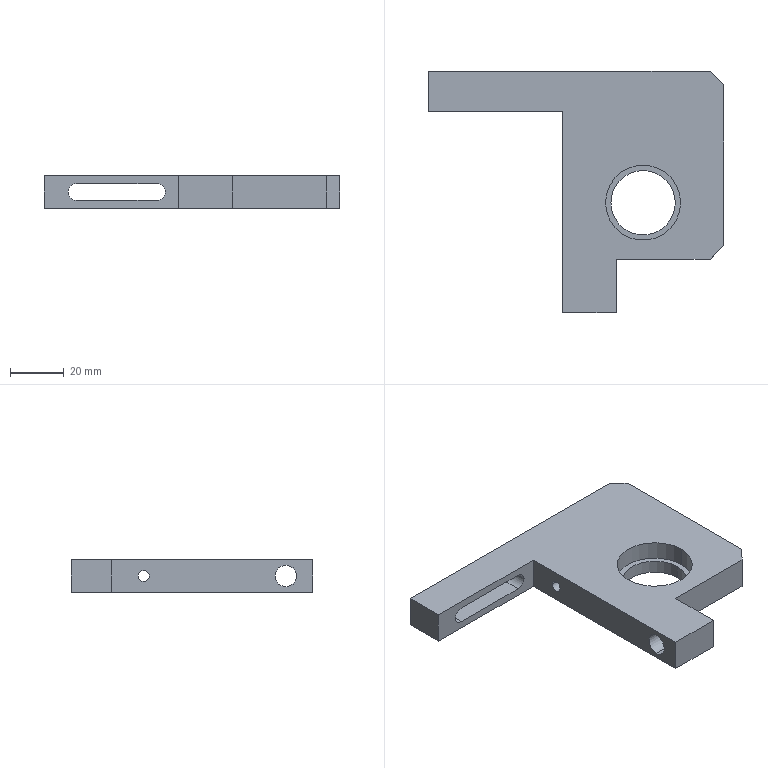Component | SolidWorks | LD101-02--Q1026-Q1-2-1 | 1 solid | 29 faces | box 110 x 90 x 12 mm | volume 49661 mm3 | plane 16 | cylinder 13 | commonest cylinder face diameters 6.2 x3 4.2 x2 10 x2 8 x2 24 x2 28 x2 | material 45
build123d program:
from build123d import *

# Parameters (mm, degrees)
SKETCH1_W           = 110
SKETCH1_H           = 90
BOSS_EXTRUDE1_DEPTH = 6
SKETCH2_W           = 50
SKETCH2_H           = 75
CUT_EXTRUDE1_DEPTH  = 107.156
SKETCH3_R           = 14
CUT_EXTRUDE2_DEPTH  = 7
SKETCH4_R           = 12
CUT_EXTRUDE3_DEPTH  = 106.707
CUT_EXTRUDE4_DEPTH  = 94.199
SKETCH6_W           = 40
SKETCH6_H           = 20
CUT_EXTRUDE5_DEPTH  = 107.156
M5_TAPPED_HOLE1_D   = 8
CHAMFER1_SIZE       = 5
SKETCH11_R          = 5
CUT_EXTRUDE6_DEPTH  = 40
M5_TAPPED_HOLE2_D   = 4.2


with BuildPart() as part:
    # Sketch1 → Boss-Extrude1 (new, symmetric)
    with BuildSketch(Plane(origin=(0, 0, 0), x_dir=(0, 0, -1), z_dir=(1, 0, 0))):
        with Locations((0, 45)):
            Rectangle(SKETCH1_W, SKETCH1_H)
    extrude(amount=BOSS_EXTRUDE1_DEPTH, both=True)

    # Sketch2 → Cut-Extrude1 (cut, through all)
    with BuildSketch(Plane(origin=(6, 0, 0), x_dir=(0, 0, -1), z_dir=(1, 0, 0))):
        with Locations((30, 52.5)):
            Rectangle(SKETCH2_W, SKETCH2_H)
    extrude(amount=-CUT_EXTRUDE1_DEPTH, mode=Mode.SUBTRACT)

    # Sketch3 → Cut-Extrude2 (cut)
    with BuildSketch(Plane.ZY.offset(-6)):
        with Locations((25, 49)):
            Circle(SKETCH3_R)
    extrude(amount=CUT_EXTRUDE2_DEPTH, mode=Mode.SUBTRACT)

    # Sketch4 → Cut-Extrude3 (cut, through all)
    with BuildSketch(Plane(origin=(-1, 0, 0), x_dir=(0, 0, -1), z_dir=(1, 0, 0))):
        with Locations((-25, 49)):
            Circle(SKETCH4_R)
    extrude(amount=-CUT_EXTRUDE3_DEPTH, mode=Mode.SUBTRACT)

    # Sketch5 → Cut-Extrude4 (cut, through all)
    with BuildSketch(Plane(origin=(0, 15, 0), x_dir=(1, 0, 0), z_dir=(0, 1, 0))):
        with BuildLine():
            Line((3.1, 43), (3.1, 13))
            ThreePointArc((3.1, 13), (0, 9.9), (-3.1, 13))
            Line((-3.1, 13), (-3.1, 43))
            ThreePointArc((-3.1, 43), (0, 46.1), (3.1, 43))
        make_face()
    extrude(amount=-CUT_EXTRUDE4_DEPTH, mode=Mode.SUBTRACT)

    # Sketch6 → Cut-Extrude5 (cut, through all)
    with BuildSketch(Plane.ZY.offset(6)):
        with Locations((35, 80)):
            Rectangle(SKETCH6_W, SKETCH6_H)
    extrude(amount=-CUT_EXTRUDE5_DEPTH, mode=Mode.SUBTRACT)

    # M5 Tapped Hole1 (through all)
    with Locations(Plane.XY.offset(15)):
        with Locations((0, 80)):
            Hole(M5_TAPPED_HOLE1_D / 2)

    # Chamfer1
    chamfer1_edges = [part.edges().sort_by_distance(p)[0] for p in [
        (0, 70, 55),
        (0, 0, 55),
    ]]
    chamfer(chamfer1_edges, length=CHAMFER1_SIZE)

    # Sketch11 → Cut-Extrude6 (cut)
    with BuildSketch(Plane.XY.offset(55)):
        with Locations((0, 27)):
            Circle(SKETCH11_R)
    extrude(amount=-CUT_EXTRUDE6_DEPTH, mode=Mode.SUBTRACT)

    # M5 Tapped Hole2 (through all)
    with Locations(Plane(origin=(0, 0, -5), x_dir=(-1, 0, 0), z_dir=(0, 0, -1))):
        with Locations((0, 27)):
            Hole(M5_TAPPED_HOLE2_D / 2)


solid = part.part

# Placed as in the assembly
solid = solid.moved(Location((346.71, -132.897, 5.257), (180, 90, 0)))
STEP:
#1=COLOUR_RGB('',0.7922,0.8196,0.9333);
#2=FILL_AREA_STYLE_COLOUR('',#1);
#3=FILL_AREA_STYLE('',(#2));
#4=SURFACE_STYLE_FILL_AREA(#3);
#5=SURFACE_SIDE_STYLE('',(#4));
#6=SURFACE_STYLE_USAGE(.BOTH.,#5);
#7=PRESENTATION_STYLE_ASSIGNMENT((#6));
#8=CARTESIAN_POINT('',(14.241,-6.378,0.207));
#9=VERTEX_POINT('',#8);
#10=CARTESIAN_POINT('',(14.241,-6.212,0.207));
#11=VERTEX_POINT('',#10);
#12=CARTESIAN_POINT('',(14.241,-6.295,0.207));
#13=DIRECTION('',(1.,0.,-0.));
#14=DIRECTION('',(0.,1.,0.));
#15=AXIS2_PLACEMENT_3D('',#12,#13,#14);
#16=CIRCLE('',#15,0.08268);
#17=EDGE_CURVE('',#9,#11,#16,.T.);
#18=ORIENTED_EDGE('',*,*,#17,.T.);
#19=CARTESIAN_POINT('',(13.453,-6.212,0.207));
#20=VERTEX_POINT('',#19);
#21=CARTESIAN_POINT('',(13.453,-6.212,0.207));
#22=DIRECTION('',(-1.,-0.,0.));
#23=VECTOR('',#22,39.37);
#24=LINE('',#21,#23);
#25=EDGE_CURVE('',#11,#20,#24,.T.);
#26=ORIENTED_EDGE('',*,*,#25,.T.);
#27=CARTESIAN_POINT('',(13.453,-6.378,0.207));
#28=VERTEX_POINT('',#27);
#29=CARTESIAN_POINT('',(13.453,-6.295,0.207));
#30=DIRECTION('',(-1.,-0.,0.));
#31=DIRECTION('',(0.,-1.,0.));
#32=AXIS2_PLACEMENT_3D('',#29,#30,#31);
#33=CIRCLE('',#32,0.08268);
#34=EDGE_CURVE('',#20,#28,#33,.T.);
#35=ORIENTED_EDGE('',*,*,#34,.T.);
#36=CARTESIAN_POINT('',(13.453,-6.378,0.207));
#37=DIRECTION('',(-1.,-0.,0.));
#38=VECTOR('',#37,39.37);
#39=LINE('',#36,#38);
#40=EDGE_CURVE('',#9,#28,#39,.T.);
#41=ORIENTED_EDGE('',*,*,#40,.F.);
#42=EDGE_LOOP('',(#18,#26,#35,#41));
#43=FACE_OUTER_BOUND('',#42,.T.);
#44=CARTESIAN_POINT('',(13.453,-6.295,0.207));
#45=DIRECTION('',(-1.,-0.,0.));
#46=DIRECTION('',(0.,-1.,0.));
#47=AXIS2_PLACEMENT_3D('',#44,#45,#46);
#48=CYLINDRICAL_SURFACE('',#47,0.08268);
#49=ADVANCED_FACE('',(#43),#48,.F.);
#50=CARTESIAN_POINT('',(14.241,-6.295,0.4038));
#51=VERTEX_POINT('',#50);
#52=CARTESIAN_POINT('',(14.241,-6.295,0.0101));
#53=VERTEX_POINT('',#52);
#54=CARTESIAN_POINT('',(14.241,-6.295,0.207));
#55=DIRECTION('',(-1.,-0.,0.));
#56=DIRECTION('',(0.,1.,0.));
#57=AXIS2_PLACEMENT_3D('',#54,#55,#56);
#58=CIRCLE('',#57,0.1969);
#59=EDGE_CURVE('',#51,#53,#58,.T.);
#60=ORIENTED_EDGE('',*,*,#59,.T.);
#61=CARTESIAN_POINT('',(15.815,-6.295,0.0101));
#62=VERTEX_POINT('',#61);
#63=CARTESIAN_POINT('',(12.896,-6.295,0.0101));
#64=DIRECTION('',(1.,0.,-0.));
#65=VECTOR('',#64,39.37);
#66=LINE('',#63,#65);
#67=EDGE_CURVE('',#53,#62,#66,.T.);
#68=ORIENTED_EDGE('',*,*,#67,.T.);
#69=CARTESIAN_POINT('',(15.815,-6.295,0.4038));
#70=VERTEX_POINT('',#69);
#71=CARTESIAN_POINT('',(15.815,-6.295,0.207));
#72=DIRECTION('',(1.,0.,-0.));
#73=DIRECTION('',(0.,0.,1.));
#74=AXIS2_PLACEMENT_3D('',#71,#72,#73);
#75=CIRCLE('',#74,0.1969);
#76=EDGE_CURVE('',#62,#70,#75,.T.);
#77=ORIENTED_EDGE('',*,*,#76,.T.);
#78=CARTESIAN_POINT('',(12.896,-6.295,0.4038));
#79=DIRECTION('',(1.,0.,-0.));
#80=VECTOR('',#79,39.37);
#81=LINE('',#78,#80);
#82=EDGE_CURVE('',#51,#70,#81,.T.);
#83=ORIENTED_EDGE('',*,*,#82,.F.);
#84=EDGE_LOOP('',(#60,#68,#77,#83));
#85=FACE_OUTER_BOUND('',#84,.T.);
#86=CARTESIAN_POINT('',(12.896,-6.295,0.207));
#87=DIRECTION('',(1.,0.,-0.));
#88=DIRECTION('',(0.,0.,1.));
#89=AXIS2_PLACEMENT_3D('',#86,#87,#88);
#90=CYLINDRICAL_SURFACE('',#89,0.1969);
#91=ADVANCED_FACE('',(#85),#90,.F.);
#92=CARTESIAN_POINT('',(13.453,-8.382,0.04947));
#93=VERTEX_POINT('',#92);
#94=CARTESIAN_POINT('',(13.453,-8.382,0.3644));
#95=VERTEX_POINT('',#94);
#96=CARTESIAN_POINT('',(13.453,-8.382,0.207));
#97=DIRECTION('',(1.,0.,-0.));
#98=DIRECTION('',(0.,1.,0.));
#99=AXIS2_PLACEMENT_3D('',#96,#97,#98);
#100=CIRCLE('',#99,0.1575);
#101=EDGE_CURVE('',#93,#95,#100,.T.);
#102=ORIENTED_EDGE('',*,*,#101,.F.);
#103=CARTESIAN_POINT('',(14.241,-8.382,0.04947));
#104=VERTEX_POINT('',#103);
#105=CARTESIAN_POINT('',(14.241,-8.382,0.04947));
#106=DIRECTION('',(1.,0.,-0.));
#107=VECTOR('',#106,39.37);
#108=LINE('',#105,#107);
#109=EDGE_CURVE('',#93,#104,#108,.T.);
#110=ORIENTED_EDGE('',*,*,#109,.T.);
#111=CARTESIAN_POINT('',(14.241,-8.382,0.3644));
#112=VERTEX_POINT('',#111);
#113=CARTESIAN_POINT('',(14.241,-8.382,0.207));
#114=DIRECTION('',(1.,0.,-0.));
#115=DIRECTION('',(0.,0.,1.));
#116=AXIS2_PLACEMENT_3D('',#113,#114,#115);
#117=CIRCLE('',#116,0.1575);
#118=EDGE_CURVE('',#104,#112,#117,.T.);
#119=ORIENTED_EDGE('',*,*,#118,.T.);
#120=CARTESIAN_POINT('',(14.241,-8.382,0.3644));
#121=DIRECTION('',(1.,0.,-0.));
#122=VECTOR('',#121,39.37);
#123=LINE('',#120,#122);
#124=EDGE_CURVE('',#95,#112,#123,.T.);
#125=ORIENTED_EDGE('',*,*,#124,.F.);
#126=EDGE_LOOP('',(#102,#110,#119,#125));
#127=FACE_OUTER_BOUND('',#126,.T.);
#128=CARTESIAN_POINT('',(14.241,-8.382,0.207));
#129=DIRECTION('',(1.,0.,-0.));
#130=DIRECTION('',(0.,0.,1.));
#131=AXIS2_PLACEMENT_3D('',#128,#129,#130);
#132=CYLINDRICAL_SURFACE('',#131,0.1575);
#133=ADVANCED_FACE('',(#127),#132,.F.);
#134=CARTESIAN_POINT('',(13.26,-5.232,0.207));
#135=VERTEX_POINT('',#134);
#136=CARTESIAN_POINT('',(13.138,-5.232,0.329));
#137=VERTEX_POINT('',#136);
#138=CARTESIAN_POINT('',(13.138,-5.232,0.207));
#139=DIRECTION('',(0.,-1.,0.));
#140=DIRECTION('',(1.,0.,0.));
#141=AXIS2_PLACEMENT_3D('',#138,#139,#140);
#142=CIRCLE('',#141,0.122);
#143=EDGE_CURVE('',#135,#137,#142,.T.);
#144=ORIENTED_EDGE('',*,*,#143,.F.);
#145=CARTESIAN_POINT('',(13.26,-5.823,0.207));
#146=VERTEX_POINT('',#145);
#147=CARTESIAN_POINT('',(13.26,-5.232,0.207));
#148=DIRECTION('',(0.,-1.,0.));
#149=VECTOR('',#148,39.37);
#150=LINE('',#147,#149);
#151=EDGE_CURVE('',#135,#146,#150,.T.);
#152=ORIENTED_EDGE('',*,*,#151,.T.);
#153=CARTESIAN_POINT('',(13.138,-5.823,0.329));
#154=VERTEX_POINT('',#153);
#155=CARTESIAN_POINT('',(13.138,-5.823,0.207));
#156=DIRECTION('',(0.,-1.,0.));
#157=DIRECTION('',(1.,0.,0.));
#158=AXIS2_PLACEMENT_3D('',#155,#156,#157);
#159=CIRCLE('',#158,0.122);
#160=EDGE_CURVE('',#146,#154,#159,.T.);
#161=ORIENTED_EDGE('',*,*,#160,.T.);
#162=CARTESIAN_POINT('',(13.138,-5.232,0.329));
#163=DIRECTION('',(0.,-1.,0.));
#164=VECTOR('',#163,39.37);
#165=LINE('',#162,#164);
#166=EDGE_CURVE('',#137,#154,#165,.T.);
#167=ORIENTED_EDGE('',*,*,#166,.F.);
#168=EDGE_LOOP('',(#144,#152,#161,#167));
#169=FACE_OUTER_BOUND('',#168,.T.);
#170=CARTESIAN_POINT('',(13.138,-5.232,0.207));
#171=DIRECTION('',(0.,-1.,0.));
#172=DIRECTION('',(1.,0.,0.));
#173=AXIS2_PLACEMENT_3D('',#170,#171,#172);
#174=CYLINDRICAL_SURFACE('',#173,0.122);
#175=ADVANCED_FACE('',(#169),#174,.F.);
#176=CARTESIAN_POINT('',(15.107,-7.161,-0.02927));
#177=VERTEX_POINT('',#176);
#178=CARTESIAN_POINT('',(14.162,-7.161,-0.02927));
#179=VERTEX_POINT('',#178);
#180=CARTESIAN_POINT('',(14.634,-7.161,-0.02927));
#181=DIRECTION('',(0.,0.,1.));
#182=DIRECTION('',(-1.,0.,0.));
#183=AXIS2_PLACEMENT_3D('',#180,#181,#182);
#184=CIRCLE('',#183,0.4724);
#185=EDGE_CURVE('',#177,#179,#184,.T.);
#186=ORIENTED_EDGE('',*,*,#185,.F.);
#187=CARTESIAN_POINT('',(15.107,-7.161,0.1676));
#188=VERTEX_POINT('',#187);
#189=CARTESIAN_POINT('',(15.107,-7.161,-0.02927));
#190=DIRECTION('',(0.,0.,1.));
#191=VECTOR('',#190,39.37);
#192=LINE('',#189,#191);
#193=EDGE_CURVE('',#177,#188,#192,.T.);
#194=ORIENTED_EDGE('',*,*,#193,.T.);
#195=CARTESIAN_POINT('',(14.162,-7.161,0.1676));
#196=VERTEX_POINT('',#195);
#197=CARTESIAN_POINT('',(14.634,-7.161,0.1676));
#198=DIRECTION('',(0.,0.,1.));
#199=DIRECTION('',(-1.,0.,0.));
#200=AXIS2_PLACEMENT_3D('',#197,#198,#199);
#201=CIRCLE('',#200,0.4724);
#202=EDGE_CURVE('',#188,#196,#201,.T.);
#203=ORIENTED_EDGE('',*,*,#202,.T.);
#204=CARTESIAN_POINT('',(14.162,-7.161,-0.02927));
#205=DIRECTION('',(0.,0.,1.));
#206=VECTOR('',#205,39.37);
#207=LINE('',#204,#206);
#208=EDGE_CURVE('',#179,#196,#207,.T.);
#209=ORIENTED_EDGE('',*,*,#208,.F.);
#210=EDGE_LOOP('',(#186,#194,#203,#209));
#211=FACE_OUTER_BOUND('',#210,.T.);
#212=CARTESIAN_POINT('',(14.634,-7.161,-0.02927));
#213=DIRECTION('',(0.,0.,1.));
#214=DIRECTION('',(-1.,0.,0.));
#215=AXIS2_PLACEMENT_3D('',#212,#213,#214);
#216=CYLINDRICAL_SURFACE('',#215,0.4724);
#217=ADVANCED_FACE('',(#211),#216,.F.);
#218=CARTESIAN_POINT('',(14.083,-7.161,0.1676));
#219=VERTEX_POINT('',#218);
#220=CARTESIAN_POINT('',(15.185,-7.161,0.1676));
#221=VERTEX_POINT('',#220);
#222=CARTESIAN_POINT('',(14.634,-7.161,0.1676));
#223=DIRECTION('',(-0.,-0.,-1.));
#224=DIRECTION('',(1.,0.,0.));
#225=AXIS2_PLACEMENT_3D('',#222,#223,#224);
#226=CIRCLE('',#225,0.5512);
#227=EDGE_CURVE('',#219,#221,#226,.T.);
#228=ORIENTED_EDGE('',*,*,#227,.T.);
#229=CARTESIAN_POINT('',(15.185,-7.161,0.4432));
#230=VERTEX_POINT('',#229);
#231=CARTESIAN_POINT('',(15.185,-7.161,0.1676));
#232=DIRECTION('',(0.,0.,1.));
#233=VECTOR('',#232,39.37);
#234=LINE('',#231,#233);
#235=EDGE_CURVE('',#221,#230,#234,.T.);
#236=ORIENTED_EDGE('',*,*,#235,.T.);
#237=CARTESIAN_POINT('',(14.083,-7.161,0.4432));
#238=VERTEX_POINT('',#237);
#239=CARTESIAN_POINT('',(14.634,-7.161,0.4432));
#240=DIRECTION('',(-0.,-0.,-1.));
#241=DIRECTION('',(1.,0.,0.));
#242=AXIS2_PLACEMENT_3D('',#239,#240,#241);
#243=CIRCLE('',#242,0.5512);
#244=EDGE_CURVE('',#238,#230,#243,.T.);
#245=ORIENTED_EDGE('',*,*,#244,.F.);
#246=CARTESIAN_POINT('',(14.083,-7.161,0.1676));
#247=DIRECTION('',(0.,0.,1.));
#248=VECTOR('',#247,39.37);
#249=LINE('',#246,#248);
#250=EDGE_CURVE('',#219,#238,#249,.T.);
#251=ORIENTED_EDGE('',*,*,#250,.F.);
#252=EDGE_LOOP('',(#228,#236,#245,#251));
#253=FACE_OUTER_BOUND('',#252,.T.);
#254=CARTESIAN_POINT('',(14.634,-7.161,0.1676));
#255=DIRECTION('',(0.,0.,1.));
#256=DIRECTION('',(-1.,0.,0.));
#257=AXIS2_PLACEMENT_3D('',#254,#255,#256);
#258=CYLINDRICAL_SURFACE('',#257,0.5512);
#259=ADVANCED_FACE('',(#253),#258,.F.);
#260=CARTESIAN_POINT('',(15.815,-7.791,0.4432));
#261=VERTEX_POINT('',#260);
#262=CARTESIAN_POINT('',(15.815,-5.429,0.4432));
#263=VERTEX_POINT('',#262);
#264=CARTESIAN_POINT('',(15.815,-5.232,0.4432));
#265=DIRECTION('',(-0.,1.,-0.));
#266=VECTOR('',#265,39.37);
#267=LINE('',#264,#266);
#268=EDGE_CURVE('',#261,#263,#267,.T.);
#269=ORIENTED_EDGE('',*,*,#268,.T.);
#270=CARTESIAN_POINT('',(15.619,-5.232,0.4432));
#271=VERTEX_POINT('',#270);
#272=CARTESIAN_POINT('',(15.619,-5.232,0.4432));
#273=DIRECTION('',(-0.7071,0.7071,0.));
#274=VECTOR('',#273,39.37);
#275=LINE('',#272,#274);
#276=EDGE_CURVE('',#263,#271,#275,.T.);
#277=ORIENTED_EDGE('',*,*,#276,.T.);
#278=CARTESIAN_POINT('',(11.485,-5.232,0.4432));
#279=VERTEX_POINT('',#278);
#280=CARTESIAN_POINT('',(15.815,-5.232,0.4432));
#281=DIRECTION('',(-1.,-0.,0.));
#282=VECTOR('',#281,39.37);
#283=LINE('',#280,#282);
#284=EDGE_CURVE('',#271,#279,#283,.T.);
#285=ORIENTED_EDGE('',*,*,#284,.T.);
#286=CARTESIAN_POINT('',(11.485,-5.823,0.4432));
#287=VERTEX_POINT('',#286);
#288=CARTESIAN_POINT('',(11.485,-5.232,0.4432));
#289=DIRECTION('',(0.,-1.,0.));
#290=VECTOR('',#289,39.37);
#291=LINE('',#288,#290);
#292=EDGE_CURVE('',#279,#287,#291,.T.);
#293=ORIENTED_EDGE('',*,*,#292,.T.);
#294=CARTESIAN_POINT('',(13.453,-5.823,0.4432));
#295=VERTEX_POINT('',#294);
#296=CARTESIAN_POINT('',(11.485,-5.823,0.4432));
#297=DIRECTION('',(-1.,-0.,0.));
#298=VECTOR('',#297,39.37);
#299=LINE('',#296,#298);
#300=EDGE_CURVE('',#295,#287,#299,.T.);
#301=ORIENTED_EDGE('',*,*,#300,.F.);
#302=CARTESIAN_POINT('',(13.453,-8.775,0.4432));
#303=VERTEX_POINT('',#302);
#304=CARTESIAN_POINT('',(13.453,-8.775,0.4432));
#305=DIRECTION('',(-0.,1.,-0.));
#306=VECTOR('',#305,39.37);
#307=LINE('',#304,#306);
#308=EDGE_CURVE('',#303,#295,#307,.T.);
#309=ORIENTED_EDGE('',*,*,#308,.F.);
#310=CARTESIAN_POINT('',(14.241,-8.775,0.4432));
#311=VERTEX_POINT('',#310);
#312=CARTESIAN_POINT('',(15.815,-8.775,0.4432));
#313=DIRECTION('',(1.,0.,-0.));
#314=VECTOR('',#313,39.37);
#315=LINE('',#312,#314);
#316=EDGE_CURVE('',#303,#311,#315,.T.);
#317=ORIENTED_EDGE('',*,*,#316,.T.);
#318=CARTESIAN_POINT('',(14.241,-7.988,0.4432));
#319=VERTEX_POINT('',#318);
#320=CARTESIAN_POINT('',(14.241,-8.775,0.4432));
#321=DIRECTION('',(0.,1.,-0.));
#322=VECTOR('',#321,39.37);
#323=LINE('',#320,#322);
#324=EDGE_CURVE('',#311,#319,#323,.T.);
#325=ORIENTED_EDGE('',*,*,#324,.T.);
#326=CARTESIAN_POINT('',(15.619,-7.988,0.4432));
#327=VERTEX_POINT('',#326);
#328=CARTESIAN_POINT('',(15.815,-7.988,0.4432));
#329=DIRECTION('',(1.,0.,-0.));
#330=VECTOR('',#329,39.37);
#331=LINE('',#328,#330);
#332=EDGE_CURVE('',#319,#327,#331,.T.);
#333=ORIENTED_EDGE('',*,*,#332,.T.);
#334=CARTESIAN_POINT('',(15.815,-7.791,0.4432));
#335=DIRECTION('',(0.7071,0.7071,-0.));
#336=VECTOR('',#335,39.37);
#337=LINE('',#334,#336);
#338=EDGE_CURVE('',#327,#261,#337,.T.);
#339=ORIENTED_EDGE('',*,*,#338,.T.);
#340=EDGE_LOOP('',(#269,#277,#285,#293,#301,#309,#317,#325,#333,#339));
#341=FACE_OUTER_BOUND('',#340,.T.);
#342=ORIENTED_EDGE('',*,*,#244,.T.);
#343=CARTESIAN_POINT('',(14.634,-7.161,0.4432));
#344=DIRECTION('',(-0.,-0.,-1.));
#345=DIRECTION('',(1.,0.,0.));
#346=AXIS2_PLACEMENT_3D('',#343,#344,#345);
#347=CIRCLE('',#346,0.5512);
#348=EDGE_CURVE('',#230,#238,#347,.T.);
#349=ORIENTED_EDGE('',*,*,#348,.T.);
#350=EDGE_LOOP('',(#342,#349));
#351=FACE_BOUND('',#350,.T.);
#352=CARTESIAN_POINT('',(13.65,-5.232,0.4432));
#353=DIRECTION('',(-0.,-0.,-1.));
#354=DIRECTION('',(1.,0.,-0.));
#355=AXIS2_PLACEMENT_3D('',#352,#353,#354);
#356=PLANE('',#355);
#357=ADVANCED_FACE('',(#341,#351),#356,.F.);
#358=CARTESIAN_POINT('',(15.815,-6.295,0.207));
#359=DIRECTION('',(1.,0.,-0.));
#360=DIRECTION('',(0.,0.,1.));
#361=AXIS2_PLACEMENT_3D('',#358,#359,#360);
#362=CIRCLE('',#361,0.1969);
#363=EDGE_CURVE('',#70,#62,#362,.T.);
#364=ORIENTED_EDGE('',*,*,#363,.F.);
#365=ORIENTED_EDGE('',*,*,#76,.F.);
#366=EDGE_LOOP('',(#364,#365));
#367=FACE_BOUND('',#366,.T.);
#368=CARTESIAN_POINT('',(15.815,-7.791,-0.02927));
#369=VERTEX_POINT('',#368);
#370=CARTESIAN_POINT('',(15.815,-5.429,-0.02927));
#371=VERTEX_POINT('',#370);
#372=CARTESIAN_POINT('',(15.815,-5.232,-0.02927));
#373=DIRECTION('',(-0.,1.,-0.));
#374=VECTOR('',#373,39.37);
#375=LINE('',#372,#374);
#376=EDGE_CURVE('',#369,#371,#375,.T.);
#377=ORIENTED_EDGE('',*,*,#376,.T.);
#378=CARTESIAN_POINT('',(15.815,-5.429,0.4432));
#379=DIRECTION('',(0.,0.,1.));
#380=VECTOR('',#379,39.37);
#381=LINE('',#378,#380);
#382=EDGE_CURVE('',#371,#263,#381,.T.);
#383=ORIENTED_EDGE('',*,*,#382,.T.);
#384=ORIENTED_EDGE('',*,*,#268,.F.);
#385=CARTESIAN_POINT('',(15.815,-7.791,0.4432));
#386=DIRECTION('',(-0.,-0.,-1.));
#387=VECTOR('',#386,39.37);
#388=LINE('',#385,#387);
#389=EDGE_CURVE('',#261,#369,#388,.T.);
#390=ORIENTED_EDGE('',*,*,#389,.T.);
#391=EDGE_LOOP('',(#377,#383,#384,#390));
#392=FACE_OUTER_BOUND('',#391,.T.);
#393=CARTESIAN_POINT('',(15.815,-5.232,0.4432));
#394=DIRECTION('',(-1.,-0.,0.));
#395=DIRECTION('',(-0.,-0.,-1.));
#396=AXIS2_PLACEMENT_3D('',#393,#394,#395);
#397=PLANE('',#396);
#398=ADVANCED_FACE('',(#367,#392),#397,.F.);
#399=CARTESIAN_POINT('',(11.957,-5.232,0.329));
#400=VERTEX_POINT('',#399);
#401=CARTESIAN_POINT('',(11.957,-5.232,0.329));
#402=DIRECTION('',(-1.,-0.,-0.));
#403=VECTOR('',#402,39.37);
#404=LINE('',#401,#403);
#405=EDGE_CURVE('',#137,#400,#404,.T.);
#406=ORIENTED_EDGE('',*,*,#405,.T.);
#407=CARTESIAN_POINT('',(11.957,-5.232,0.08491));
#408=VERTEX_POINT('',#407);
#409=CARTESIAN_POINT('',(11.957,-5.232,0.207));
#410=DIRECTION('',(0.,-1.,0.));
#411=DIRECTION('',(1.,0.,0.));
#412=AXIS2_PLACEMENT_3D('',#409,#410,#411);
#413=CIRCLE('',#412,0.122);
#414=EDGE_CURVE('',#400,#408,#413,.T.);
#415=ORIENTED_EDGE('',*,*,#414,.T.);
#416=CARTESIAN_POINT('',(13.138,-5.232,0.08491));
#417=VERTEX_POINT('',#416);
#418=CARTESIAN_POINT('',(11.957,-5.232,0.08491));
#419=DIRECTION('',(1.,0.,0.));
#420=VECTOR('',#419,39.37);
#421=LINE('',#418,#420);
#422=EDGE_CURVE('',#408,#417,#421,.T.);
#423=ORIENTED_EDGE('',*,*,#422,.T.);
#424=CARTESIAN_POINT('',(13.138,-5.232,0.207));
#425=DIRECTION('',(0.,-1.,0.));
#426=DIRECTION('',(1.,0.,0.));
#427=AXIS2_PLACEMENT_3D('',#424,#425,#426);
#428=CIRCLE('',#427,0.122);
#429=EDGE_CURVE('',#417,#135,#428,.T.);
#430=ORIENTED_EDGE('',*,*,#429,.T.);
#431=ORIENTED_EDGE('',*,*,#143,.T.);
#432=EDGE_LOOP('',(#406,#415,#423,#430,#431));
#433=FACE_BOUND('',#432,.T.);
#434=ORIENTED_EDGE('',*,*,#284,.F.);
#435=CARTESIAN_POINT('',(15.619,-5.232,-0.02927));
#436=VERTEX_POINT('',#435);
#437=CARTESIAN_POINT('',(15.619,-5.232,0.4432));
#438=DIRECTION('',(-0.,-0.,-1.));
#439=VECTOR('',#438,39.37);
#440=LINE('',#437,#439);
#441=EDGE_CURVE('',#271,#436,#440,.T.);
#442=ORIENTED_EDGE('',*,*,#441,.T.);
#443=CARTESIAN_POINT('',(11.485,-5.232,-0.02927));
#444=VERTEX_POINT('',#443);
#445=CARTESIAN_POINT('',(15.815,-5.232,-0.02927));
#446=DIRECTION('',(-1.,-0.,0.));
#447=VECTOR('',#446,39.37);
#448=LINE('',#445,#447);
#449=EDGE_CURVE('',#436,#444,#448,.T.);
#450=ORIENTED_EDGE('',*,*,#449,.T.);
#451=CARTESIAN_POINT('',(11.485,-5.232,0.4432));
#452=DIRECTION('',(-0.,-0.,-1.));
#453=VECTOR('',#452,39.37);
#454=LINE('',#451,#453);
#455=EDGE_CURVE('',#279,#444,#454,.T.);
#456=ORIENTED_EDGE('',*,*,#455,.F.);
#457=EDGE_LOOP('',(#434,#442,#450,#456));
#458=FACE_OUTER_BOUND('',#457,.T.);
#459=CARTESIAN_POINT('',(15.815,-5.232,0.4432));
#460=DIRECTION('',(0.,-1.,0.));
#461=DIRECTION('',(1.,0.,-0.));
#462=AXIS2_PLACEMENT_3D('',#459,#460,#461);
#463=PLANE('',#462);
#464=ADVANCED_FACE('',(#433,#458),#463,.F.);
#465=CARTESIAN_POINT('',(11.485,-5.823,-0.02927));
#466=VERTEX_POINT('',#465);
#467=CARTESIAN_POINT('',(11.485,-5.232,-0.02927));
#468=DIRECTION('',(0.,-1.,0.));
#469=VECTOR('',#468,39.37);
#470=LINE('',#467,#469);
#471=EDGE_CURVE('',#444,#466,#470,.T.);
#472=ORIENTED_EDGE('',*,*,#471,.T.);
#473=CARTESIAN_POINT('',(11.485,-5.823,-0.02927));
#474=DIRECTION('',(0.,0.,1.));
#475=VECTOR('',#474,39.37);
#476=LINE('',#473,#475);
#477=EDGE_CURVE('',#466,#287,#476,.T.);
#478=ORIENTED_EDGE('',*,*,#477,.T.);
#479=ORIENTED_EDGE('',*,*,#292,.F.);
#480=ORIENTED_EDGE('',*,*,#455,.T.);
#481=EDGE_LOOP('',(#472,#478,#479,#480));
#482=FACE_OUTER_BOUND('',#481,.T.);
#483=CARTESIAN_POINT('',(11.485,-5.232,0.4432));
#484=DIRECTION('',(1.,0.,-0.));
#485=DIRECTION('',(0.,0.,1.));
#486=AXIS2_PLACEMENT_3D('',#483,#484,#485);
#487=PLANE('',#486);
#488=ADVANCED_FACE('',(#482),#487,.F.);
#489=CARTESIAN_POINT('',(13.453,-8.775,-0.02927));
#490=VERTEX_POINT('',#489);
#491=CARTESIAN_POINT('',(14.241,-8.775,-0.02927));
#492=VERTEX_POINT('',#491);
#493=CARTESIAN_POINT('',(15.815,-8.775,-0.02927));
#494=DIRECTION('',(1.,0.,-0.));
#495=VECTOR('',#494,39.37);
#496=LINE('',#493,#495);
#497=EDGE_CURVE('',#490,#492,#496,.T.);
#498=ORIENTED_EDGE('',*,*,#497,.T.);
#499=CARTESIAN_POINT('',(14.241,-8.775,0.4432));
#500=DIRECTION('',(-0.,-0.,-1.));
#501=VECTOR('',#500,39.37);
#502=LINE('',#499,#501);
#503=EDGE_CURVE('',#311,#492,#502,.T.);
#504=ORIENTED_EDGE('',*,*,#503,.F.);
#505=ORIENTED_EDGE('',*,*,#316,.F.);
#506=CARTESIAN_POINT('',(13.453,-8.775,-0.02927));
#507=DIRECTION('',(0.,0.,1.));
#508=VECTOR('',#507,39.37);
#509=LINE('',#506,#508);
#510=EDGE_CURVE('',#490,#303,#509,.T.);
#511=ORIENTED_EDGE('',*,*,#510,.F.);
#512=EDGE_LOOP('',(#498,#504,#505,#511));
#513=FACE_OUTER_BOUND('',#512,.T.);
#514=CARTESIAN_POINT('',(15.815,-8.775,0.4432));
#515=DIRECTION('',(-0.,1.,-0.));
#516=DIRECTION('',(-1.,-0.,0.));
#517=AXIS2_PLACEMENT_3D('',#514,#515,#516);
#518=PLANE('',#517);
#519=ADVANCED_FACE('',(#513),#518,.F.);
#520=ORIENTED_EDGE('',*,*,#449,.F.);
#521=CARTESIAN_POINT('',(14.634,-4.248,-0.02927));
#522=DIRECTION('',(0.7071,-0.7071,-0.));
#523=VECTOR('',#522,39.37);
#524=LINE('',#521,#523);
#525=EDGE_CURVE('',#436,#371,#524,.T.);
#526=ORIENTED_EDGE('',*,*,#525,.T.);
#527=ORIENTED_EDGE('',*,*,#376,.F.);
#528=CARTESIAN_POINT('',(15.619,-7.988,-0.02927));
#529=VERTEX_POINT('',#528);
#530=CARTESIAN_POINT('',(16.012,-7.594,-0.02927));
#531=DIRECTION('',(-0.7071,-0.7071,0.));
#532=VECTOR('',#531,39.37);
#533=LINE('',#530,#532);
#534=EDGE_CURVE('',#369,#529,#533,.T.);
#535=ORIENTED_EDGE('',*,*,#534,.T.);
#536=CARTESIAN_POINT('',(14.241,-7.988,-0.02927));
#537=VERTEX_POINT('',#536);
#538=CARTESIAN_POINT('',(15.815,-7.988,-0.02927));
#539=DIRECTION('',(1.,0.,-0.));
#540=VECTOR('',#539,39.37);
#541=LINE('',#538,#540);
#542=EDGE_CURVE('',#537,#529,#541,.T.);
#543=ORIENTED_EDGE('',*,*,#542,.F.);
#544=CARTESIAN_POINT('',(14.241,-8.775,-0.02927));
#545=DIRECTION('',(0.,1.,-0.));
#546=VECTOR('',#545,39.37);
#547=LINE('',#544,#546);
#548=EDGE_CURVE('',#492,#537,#547,.T.);
#549=ORIENTED_EDGE('',*,*,#548,.F.);
#550=ORIENTED_EDGE('',*,*,#497,.F.);
#551=CARTESIAN_POINT('',(13.453,-5.823,-0.02927));
#552=VERTEX_POINT('',#551);
#553=CARTESIAN_POINT('',(13.453,-8.775,-0.02927));
#554=DIRECTION('',(-0.,1.,-0.));
#555=VECTOR('',#554,39.37);
#556=LINE('',#553,#555);
#557=EDGE_CURVE('',#490,#552,#556,.T.);
#558=ORIENTED_EDGE('',*,*,#557,.T.);
#559=CARTESIAN_POINT('',(11.485,-5.823,-0.02927));
#560=DIRECTION('',(-1.,-0.,0.));
#561=VECTOR('',#560,39.37);
#562=LINE('',#559,#561);
#563=EDGE_CURVE('',#552,#466,#562,.T.);
#564=ORIENTED_EDGE('',*,*,#563,.T.);
#565=ORIENTED_EDGE('',*,*,#471,.F.);
#566=EDGE_LOOP('',(#520,#526,#527,#535,#543,#549,#550,#558,#564,#565));
#567=FACE_OUTER_BOUND('',#566,.T.);
#568=CARTESIAN_POINT('',(14.634,-7.161,-0.02927));
#569=DIRECTION('',(0.,0.,1.));
#570=DIRECTION('',(-1.,0.,0.));
#571=AXIS2_PLACEMENT_3D('',#568,#569,#570);
#572=CIRCLE('',#571,0.4724);
#573=EDGE_CURVE('',#179,#177,#572,.T.);
#574=ORIENTED_EDGE('',*,*,#573,.T.);
#575=ORIENTED_EDGE('',*,*,#185,.T.);
#576=EDGE_LOOP('',(#574,#575));
#577=FACE_BOUND('',#576,.T.);
#578=CARTESIAN_POINT('',(13.65,-5.232,-0.02927));
#579=DIRECTION('',(-0.,-0.,-1.));
#580=DIRECTION('',(1.,0.,-0.));
#581=AXIS2_PLACEMENT_3D('',#578,#579,#580);
#582=PLANE('',#581);
#583=ADVANCED_FACE('',(#567,#577),#582,.T.);
#584=CARTESIAN_POINT('',(11.957,-5.823,0.08491));
#585=VERTEX_POINT('',#584);
#586=CARTESIAN_POINT('',(13.138,-5.823,0.08491));
#587=VERTEX_POINT('',#586);
#588=CARTESIAN_POINT('',(11.957,-5.823,0.08491));
#589=DIRECTION('',(1.,0.,0.));
#590=VECTOR('',#589,39.37);
#591=LINE('',#588,#590);
#592=EDGE_CURVE('',#585,#587,#591,.T.);
#593=ORIENTED_EDGE('',*,*,#592,.F.);
#594=CARTESIAN_POINT('',(11.957,-5.823,0.329));
#595=VERTEX_POINT('',#594);
#596=CARTESIAN_POINT('',(11.957,-5.823,0.207));
#597=DIRECTION('',(0.,-1.,0.));
#598=DIRECTION('',(1.,0.,0.));
#599=AXIS2_PLACEMENT_3D('',#596,#597,#598);
#600=CIRCLE('',#599,0.122);
#601=EDGE_CURVE('',#595,#585,#600,.T.);
#602=ORIENTED_EDGE('',*,*,#601,.F.);
#603=CARTESIAN_POINT('',(11.957,-5.823,0.329));
#604=DIRECTION('',(-1.,-0.,-0.));
#605=VECTOR('',#604,39.37);
#606=LINE('',#603,#605);
#607=EDGE_CURVE('',#154,#595,#606,.T.);
#608=ORIENTED_EDGE('',*,*,#607,.F.);
#609=ORIENTED_EDGE('',*,*,#160,.F.);
#610=CARTESIAN_POINT('',(13.138,-5.823,0.207));
#611=DIRECTION('',(0.,-1.,0.));
#612=DIRECTION('',(1.,0.,0.));
#613=AXIS2_PLACEMENT_3D('',#610,#611,#612);
#614=CIRCLE('',#613,0.122);
#615=EDGE_CURVE('',#587,#146,#614,.T.);
#616=ORIENTED_EDGE('',*,*,#615,.F.);
#617=EDGE_LOOP('',(#593,#602,#608,#609,#616));
#618=FACE_BOUND('',#617,.T.);
#619=ORIENTED_EDGE('',*,*,#300,.T.);
#620=ORIENTED_EDGE('',*,*,#477,.F.);
#621=ORIENTED_EDGE('',*,*,#563,.F.);
#622=CARTESIAN_POINT('',(13.453,-5.823,-0.02927));
#623=DIRECTION('',(0.,0.,1.));
#624=VECTOR('',#623,39.37);
#625=LINE('',#622,#624);
#626=EDGE_CURVE('',#552,#295,#625,.T.);
#627=ORIENTED_EDGE('',*,*,#626,.T.);
#628=EDGE_LOOP('',(#619,#620,#621,#627));
#629=FACE_OUTER_BOUND('',#628,.T.);
#630=CARTESIAN_POINT('',(11.485,-5.823,-0.02927));
#631=DIRECTION('',(-0.,1.,-0.));
#632=DIRECTION('',(-1.,-0.,0.));
#633=AXIS2_PLACEMENT_3D('',#630,#631,#632);
#634=PLANE('',#633);
#635=ADVANCED_FACE('',(#618,#629),#634,.F.);
#636=CARTESIAN_POINT('',(13.453,-6.295,0.207));
#637=DIRECTION('',(-1.,-0.,0.));
#638=DIRECTION('',(0.,-1.,0.));
#639=AXIS2_PLACEMENT_3D('',#636,#637,#638);
#640=CIRCLE('',#639,0.08268);
#641=EDGE_CURVE('',#28,#20,#640,.T.);
#642=ORIENTED_EDGE('',*,*,#641,.F.);
#643=ORIENTED_EDGE('',*,*,#34,.F.);
#644=EDGE_LOOP('',(#642,#643));
#645=FACE_BOUND('',#644,.T.);
#646=CARTESIAN_POINT('',(13.453,-8.382,0.207));
#647=DIRECTION('',(1.,0.,-0.));
#648=DIRECTION('',(0.,1.,0.));
#649=AXIS2_PLACEMENT_3D('',#646,#647,#648);
#650=CIRCLE('',#649,0.1575);
#651=EDGE_CURVE('',#95,#93,#650,.T.);
#652=ORIENTED_EDGE('',*,*,#651,.T.);
#653=ORIENTED_EDGE('',*,*,#101,.T.);
#654=EDGE_LOOP('',(#652,#653));
#655=FACE_BOUND('',#654,.T.);
#656=ORIENTED_EDGE('',*,*,#308,.T.);
#657=ORIENTED_EDGE('',*,*,#626,.F.);
#658=ORIENTED_EDGE('',*,*,#557,.F.);
#659=ORIENTED_EDGE('',*,*,#510,.T.);
#660=EDGE_LOOP('',(#656,#657,#658,#659));
#661=FACE_OUTER_BOUND('',#660,.T.);
#662=CARTESIAN_POINT('',(13.453,-8.775,-0.02927));
#663=DIRECTION('',(1.,0.,-0.));
#664=DIRECTION('',(-0.,1.,-0.));
#665=AXIS2_PLACEMENT_3D('',#662,#663,#664);
#666=PLANE('',#665);
#667=ADVANCED_FACE('',(#645,#655,#661),#666,.F.);
#668=ORIENTED_EDGE('',*,*,#235,.F.);
#669=CARTESIAN_POINT('',(14.634,-7.161,0.1676));
#670=DIRECTION('',(-0.,-0.,-1.));
#671=DIRECTION('',(1.,0.,0.));
#672=AXIS2_PLACEMENT_3D('',#669,#670,#671);
#673=CIRCLE('',#672,0.5512);
#674=EDGE_CURVE('',#221,#219,#673,.T.);
#675=ORIENTED_EDGE('',*,*,#674,.T.);
#676=ORIENTED_EDGE('',*,*,#250,.T.);
#677=ORIENTED_EDGE('',*,*,#348,.F.);
#678=EDGE_LOOP('',(#668,#675,#676,#677));
#679=FACE_OUTER_BOUND('',#678,.T.);
#680=CARTESIAN_POINT('',(14.634,-7.161,0.1676));
#681=DIRECTION('',(0.,0.,1.));
#682=DIRECTION('',(-1.,0.,0.));
#683=AXIS2_PLACEMENT_3D('',#680,#681,#682);
#684=CYLINDRICAL_SURFACE('',#683,0.5512);
#685=ADVANCED_FACE('',(#679),#684,.F.);
#686=CARTESIAN_POINT('',(14.634,-7.161,0.1676));
#687=DIRECTION('',(0.,0.,1.));
#688=DIRECTION('',(-1.,0.,0.));
#689=AXIS2_PLACEMENT_3D('',#686,#687,#688);
#690=CIRCLE('',#689,0.4724);
#691=EDGE_CURVE('',#196,#188,#690,.T.);
#692=ORIENTED_EDGE('',*,*,#691,.F.);
#693=ORIENTED_EDGE('',*,*,#202,.F.);
#694=EDGE_LOOP('',(#692,#693));
#695=FACE_BOUND('',#694,.T.);
#696=ORIENTED_EDGE('',*,*,#227,.F.);
#697=ORIENTED_EDGE('',*,*,#674,.F.);
#698=EDGE_LOOP('',(#696,#697));
#699=FACE_OUTER_BOUND('',#698,.T.);
#700=CARTESIAN_POINT('',(14.634,-7.161,0.1676));
#701=DIRECTION('',(-0.,-0.,-1.));
#702=DIRECTION('',(1.,0.,-0.));
#703=AXIS2_PLACEMENT_3D('',#700,#701,#702);
#704=PLANE('',#703);
#705=ADVANCED_FACE('',(#695,#699),#704,.F.);
#706=ORIENTED_EDGE('',*,*,#193,.F.);
#707=ORIENTED_EDGE('',*,*,#573,.F.);
#708=ORIENTED_EDGE('',*,*,#208,.T.);
#709=ORIENTED_EDGE('',*,*,#691,.T.);
#710=EDGE_LOOP('',(#706,#707,#708,#709));
#711=FACE_OUTER_BOUND('',#710,.T.);
#712=CARTESIAN_POINT('',(14.634,-7.161,-0.02927));
#713=DIRECTION('',(0.,0.,1.));
#714=DIRECTION('',(-1.,0.,0.));
#715=AXIS2_PLACEMENT_3D('',#712,#713,#714);
#716=CYLINDRICAL_SURFACE('',#715,0.4724);
#717=ADVANCED_FACE('',(#711),#716,.F.);
#718=ORIENTED_EDGE('',*,*,#601,.T.);
#719=CARTESIAN_POINT('',(11.957,-5.232,0.08491));
#720=DIRECTION('',(0.,-1.,0.));
#721=VECTOR('',#720,39.37);
#722=LINE('',#719,#721);
#723=EDGE_CURVE('',#408,#585,#722,.T.);
#724=ORIENTED_EDGE('',*,*,#723,.F.);
#725=ORIENTED_EDGE('',*,*,#414,.F.);
#726=CARTESIAN_POINT('',(11.957,-5.232,0.329));
#727=DIRECTION('',(0.,-1.,0.));
#728=VECTOR('',#727,39.37);
#729=LINE('',#726,#728);
#730=EDGE_CURVE('',#400,#595,#729,.T.);
#731=ORIENTED_EDGE('',*,*,#730,.T.);
#732=EDGE_LOOP('',(#718,#724,#725,#731));
#733=FACE_OUTER_BOUND('',#732,.T.);
#734=CARTESIAN_POINT('',(11.957,-5.232,0.207));
#735=DIRECTION('',(0.,-1.,0.));
#736=DIRECTION('',(1.,0.,0.));
#737=AXIS2_PLACEMENT_3D('',#734,#735,#736);
#738=CYLINDRICAL_SURFACE('',#737,0.122);
#739=ADVANCED_FACE('',(#733),#738,.F.);
#740=ORIENTED_EDGE('',*,*,#607,.T.);
#741=ORIENTED_EDGE('',*,*,#730,.F.);
#742=ORIENTED_EDGE('',*,*,#405,.F.);
#743=ORIENTED_EDGE('',*,*,#166,.T.);
#744=EDGE_LOOP('',(#740,#741,#742,#743));
#745=FACE_OUTER_BOUND('',#744,.T.);
#746=CARTESIAN_POINT('',(11.957,-5.232,0.329));
#747=DIRECTION('',(-0.,-0.,1.));
#748=DIRECTION('',(-1.,-0.,-0.));
#749=AXIS2_PLACEMENT_3D('',#746,#747,#748);
#750=PLANE('',#749);
#751=ADVANCED_FACE('',(#745),#750,.F.);
#752=ORIENTED_EDGE('',*,*,#151,.F.);
#753=ORIENTED_EDGE('',*,*,#429,.F.);
#754=CARTESIAN_POINT('',(13.138,-5.232,0.08491));
#755=DIRECTION('',(0.,-1.,0.));
#756=VECTOR('',#755,39.37);
#757=LINE('',#754,#756);
#758=EDGE_CURVE('',#417,#587,#757,.T.);
#759=ORIENTED_EDGE('',*,*,#758,.T.);
#760=ORIENTED_EDGE('',*,*,#615,.T.);
#761=EDGE_LOOP('',(#752,#753,#759,#760));
#762=FACE_OUTER_BOUND('',#761,.T.);
#763=CARTESIAN_POINT('',(13.138,-5.232,0.207));
#764=DIRECTION('',(0.,-1.,0.));
#765=DIRECTION('',(1.,0.,0.));
#766=AXIS2_PLACEMENT_3D('',#763,#764,#765);
#767=CYLINDRICAL_SURFACE('',#766,0.122);
#768=ADVANCED_FACE('',(#762),#767,.F.);
#769=ORIENTED_EDGE('',*,*,#592,.T.);
#770=ORIENTED_EDGE('',*,*,#758,.F.);
#771=ORIENTED_EDGE('',*,*,#422,.F.);
#772=ORIENTED_EDGE('',*,*,#723,.T.);
#773=EDGE_LOOP('',(#769,#770,#771,#772));
#774=FACE_OUTER_BOUND('',#773,.T.);
#775=CARTESIAN_POINT('',(11.957,-5.232,0.08491));
#776=DIRECTION('',(0.,0.,-1.));
#777=DIRECTION('',(1.,0.,0.));
#778=AXIS2_PLACEMENT_3D('',#775,#776,#777);
#779=PLANE('',#778);
#780=ADVANCED_FACE('',(#774),#779,.F.);
#781=ORIENTED_EDGE('',*,*,#542,.T.);
#782=CARTESIAN_POINT('',(15.619,-7.988,0.4432));
#783=DIRECTION('',(0.,0.,1.));
#784=VECTOR('',#783,39.37);
#785=LINE('',#782,#784);
#786=EDGE_CURVE('',#529,#327,#785,.T.);
#787=ORIENTED_EDGE('',*,*,#786,.T.);
#788=ORIENTED_EDGE('',*,*,#332,.F.);
#789=CARTESIAN_POINT('',(14.241,-7.988,0.4432));
#790=DIRECTION('',(-0.,-0.,-1.));
#791=VECTOR('',#790,39.37);
#792=LINE('',#789,#791);
#793=EDGE_CURVE('',#319,#537,#792,.T.);
#794=ORIENTED_EDGE('',*,*,#793,.T.);
#795=EDGE_LOOP('',(#781,#787,#788,#794));
#796=FACE_OUTER_BOUND('',#795,.T.);
#797=CARTESIAN_POINT('',(15.815,-7.988,0.4432));
#798=DIRECTION('',(-0.,1.,-0.));
#799=DIRECTION('',(-1.,-0.,0.));
#800=AXIS2_PLACEMENT_3D('',#797,#798,#799);
#801=PLANE('',#800);
#802=ADVANCED_FACE('',(#796),#801,.F.);
#803=CARTESIAN_POINT('',(14.241,-8.382,0.207));
#804=DIRECTION('',(1.,0.,-0.));
#805=DIRECTION('',(0.,0.,1.));
#806=AXIS2_PLACEMENT_3D('',#803,#804,#805);
#807=CIRCLE('',#806,0.1575);
#808=EDGE_CURVE('',#112,#104,#807,.T.);
#809=ORIENTED_EDGE('',*,*,#808,.F.);
#810=ORIENTED_EDGE('',*,*,#118,.F.);
#811=EDGE_LOOP('',(#809,#810));
#812=FACE_BOUND('',#811,.T.);
#813=ORIENTED_EDGE('',*,*,#548,.T.);
#814=ORIENTED_EDGE('',*,*,#793,.F.);
#815=ORIENTED_EDGE('',*,*,#324,.F.);
#816=ORIENTED_EDGE('',*,*,#503,.T.);
#817=EDGE_LOOP('',(#813,#814,#815,#816));
#818=FACE_OUTER_BOUND('',#817,.T.);
#819=CARTESIAN_POINT('',(14.241,-8.775,0.4432));
#820=DIRECTION('',(-1.,0.,0.));
#821=DIRECTION('',(-0.,-1.,0.));
#822=AXIS2_PLACEMENT_3D('',#819,#820,#821);
#823=PLANE('',#822);
#824=ADVANCED_FACE('',(#812,#818),#823,.F.);
#825=ORIENTED_EDGE('',*,*,#109,.F.);
#826=ORIENTED_EDGE('',*,*,#651,.F.);
#827=ORIENTED_EDGE('',*,*,#124,.T.);
#828=ORIENTED_EDGE('',*,*,#808,.T.);
#829=EDGE_LOOP('',(#825,#826,#827,#828));
#830=FACE_OUTER_BOUND('',#829,.T.);
#831=CARTESIAN_POINT('',(14.241,-8.382,0.207));
#832=DIRECTION('',(1.,0.,-0.));
#833=DIRECTION('',(0.,0.,1.));
#834=AXIS2_PLACEMENT_3D('',#831,#832,#833);
#835=CYLINDRICAL_SURFACE('',#834,0.1575);
#836=ADVANCED_FACE('',(#830),#835,.F.);
#837=ORIENTED_EDGE('',*,*,#276,.F.);
#838=ORIENTED_EDGE('',*,*,#382,.F.);
#839=ORIENTED_EDGE('',*,*,#525,.F.);
#840=ORIENTED_EDGE('',*,*,#441,.F.);
#841=EDGE_LOOP('',(#837,#838,#839,#840));
#842=FACE_OUTER_BOUND('',#841,.T.);
#843=CARTESIAN_POINT('',(15.619,-5.232,0.4432));
#844=DIRECTION('',(-0.7071,-0.7071,0.));
#845=DIRECTION('',(-0.,-0.,-1.));
#846=AXIS2_PLACEMENT_3D('',#843,#844,#845);
#847=PLANE('',#846);
#848=ADVANCED_FACE('',(#842),#847,.F.);
#849=ORIENTED_EDGE('',*,*,#338,.F.);
#850=ORIENTED_EDGE('',*,*,#786,.F.);
#851=ORIENTED_EDGE('',*,*,#534,.F.);
#852=ORIENTED_EDGE('',*,*,#389,.F.);
#853=EDGE_LOOP('',(#849,#850,#851,#852));
#854=FACE_OUTER_BOUND('',#853,.T.);
#855=CARTESIAN_POINT('',(15.815,-7.791,0.4432));
#856=DIRECTION('',(-0.7071,0.7071,0.));
#857=DIRECTION('',(-0.,-0.,-1.));
#858=AXIS2_PLACEMENT_3D('',#855,#856,#857);
#859=PLANE('',#858);
#860=ADVANCED_FACE('',(#854),#859,.F.);
#861=ORIENTED_EDGE('',*,*,#67,.F.);
#862=CARTESIAN_POINT('',(14.241,-6.295,0.207));
#863=DIRECTION('',(-1.,-0.,0.));
#864=DIRECTION('',(0.,1.,0.));
#865=AXIS2_PLACEMENT_3D('',#862,#863,#864);
#866=CIRCLE('',#865,0.1969);
#867=EDGE_CURVE('',#53,#51,#866,.T.);
#868=ORIENTED_EDGE('',*,*,#867,.T.);
#869=ORIENTED_EDGE('',*,*,#82,.T.);
#870=ORIENTED_EDGE('',*,*,#363,.T.);
#871=EDGE_LOOP('',(#861,#868,#869,#870));
#872=FACE_OUTER_BOUND('',#871,.T.);
#873=CARTESIAN_POINT('',(12.896,-6.295,0.207));
#874=DIRECTION('',(1.,0.,-0.));
#875=DIRECTION('',(0.,0.,1.));
#876=AXIS2_PLACEMENT_3D('',#873,#874,#875);
#877=CYLINDRICAL_SURFACE('',#876,0.1969);
#878=ADVANCED_FACE('',(#872),#877,.F.);
#879=ORIENTED_EDGE('',*,*,#17,.F.);
#880=CARTESIAN_POINT('',(14.241,-6.295,0.207));
#881=DIRECTION('',(1.,0.,-0.));
#882=DIRECTION('',(0.,1.,0.));
#883=AXIS2_PLACEMENT_3D('',#880,#881,#882);
#884=CIRCLE('',#883,0.08268);
#885=EDGE_CURVE('',#11,#9,#884,.T.);
#886=ORIENTED_EDGE('',*,*,#885,.F.);
#887=EDGE_LOOP('',(#879,#886));
#888=FACE_BOUND('',#887,.T.);
#889=ORIENTED_EDGE('',*,*,#59,.F.);
#890=ORIENTED_EDGE('',*,*,#867,.F.);
#891=EDGE_LOOP('',(#889,#890));
#892=FACE_OUTER_BOUND('',#891,.T.);
#893=CARTESIAN_POINT('',(14.241,-8.775,-0.02927));
#894=DIRECTION('',(1.,0.,-0.));
#895=DIRECTION('',(-0.,1.,-0.));
#896=AXIS2_PLACEMENT_3D('',#893,#894,#895);
#897=PLANE('',#896);
#898=ADVANCED_FACE('',(#888,#892),#897,.T.);
#899=ORIENTED_EDGE('',*,*,#25,.F.);
#900=ORIENTED_EDGE('',*,*,#885,.T.);
#901=ORIENTED_EDGE('',*,*,#40,.T.);
#902=ORIENTED_EDGE('',*,*,#641,.T.);
#903=EDGE_LOOP('',(#899,#900,#901,#902));
#904=FACE_OUTER_BOUND('',#903,.T.);
#905=CARTESIAN_POINT('',(13.453,-6.295,0.207));
#906=DIRECTION('',(-1.,-0.,0.));
#907=DIRECTION('',(0.,-1.,0.));
#908=AXIS2_PLACEMENT_3D('',#905,#906,#907);
#909=CYLINDRICAL_SURFACE('',#908,0.08268);
#910=ADVANCED_FACE('',(#904),#909,.F.);
#911=CLOSED_SHELL('',(#49,#91,#133,#175,#217,#259,#357,#398,#464,#488,#519,#583,#635,#667,#685,#705,#717,#739,#751,#768,#780,#802,#824,#836,#848,#860,#878,#898,#910));
#912=MANIFOLD_SOLID_BREP('',#911);
#913=STYLED_ITEM('',(#7),#912);
#914=PRESENTATION_LAYER_ASSIGNMENT('','',(#913));
#915=CARTESIAN_POINT('',(0.,0.,0.));
#916=DIRECTION('',(0.,0.,1.));
#917=DIRECTION('',(1.,0.,0.));
#918=AXIS2_PLACEMENT_3D('',#915,#916,#917);
#919=(LENGTH_UNIT()NAMED_UNIT(*)SI_UNIT($,.METRE.));
#920=LENGTH_MEASURE_WITH_UNIT(LENGTH_MEASURE(0.0254),#919);
#921=DIMENSIONAL_EXPONENTS(1.,0.,0.,0.,0.,0.,0.);
#922=(CONVERSION_BASED_UNIT('',#920)LENGTH_UNIT()NAMED_UNIT(#921));
#923=UNCERTAINTY_MEASURE_WITH_UNIT(LENGTH_MEASURE(0.00001),#922,'','');
#924=(NAMED_UNIT(*)PLANE_ANGLE_UNIT()SI_UNIT($,.RADIAN.));
#925=(NAMED_UNIT(*)SI_UNIT($,.STERADIAN.)SOLID_ANGLE_UNIT());
#926=(GEOMETRIC_REPRESENTATION_CONTEXT(3)GLOBAL_UNCERTAINTY_ASSIGNED_CONTEXT((#923))GLOBAL_UNIT_ASSIGNED_CONTEXT((#922,#924,#925))REPRESENTATION_CONTEXT('',''));
#927=ADVANCED_BREP_SHAPE_REPRESENTATION('',(#912,#918),#926);
#928=(LENGTH_UNIT()NAMED_UNIT(*)SI_UNIT($,.METRE.));
#929=LENGTH_MEASURE_WITH_UNIT(LENGTH_MEASURE(0.0254),#928);
#930=DIMENSIONAL_EXPONENTS(1.,0.,0.,0.,0.,0.,0.);
#931=(CONVERSION_BASED_UNIT('',#929)LENGTH_UNIT()NAMED_UNIT(#930));
#932=UNCERTAINTY_MEASURE_WITH_UNIT(LENGTH_MEASURE(0.00001),#931,'','');
#933=(NAMED_UNIT(*)PLANE_ANGLE_UNIT()SI_UNIT($,.RADIAN.));
#934=(NAMED_UNIT(*)SI_UNIT($,.STERADIAN.)SOLID_ANGLE_UNIT());
#935=(GEOMETRIC_REPRESENTATION_CONTEXT(3)GLOBAL_UNCERTAINTY_ASSIGNED_CONTEXT((#932))GLOBAL_UNIT_ASSIGNED_CONTEXT((#931,#933,#934))REPRESENTATION_CONTEXT('',''));
#936=MECHANICAL_DESIGN_GEOMETRIC_PRESENTATION_REPRESENTATION('',(#913),#935);